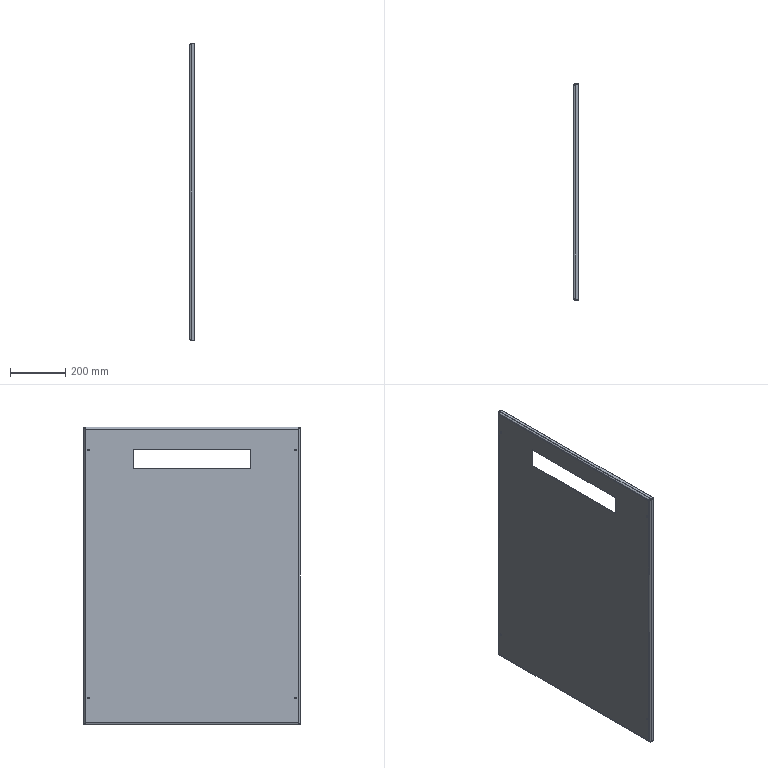Component | SolidWorks | RearLowerDoorPanel(No.28)-1 | 1 solid | 50 faces | volume 1733113 mm3 | plane 26 | cylinder 16 | spline 8 | commonest cylinder face diameters 6.5 x8 14 x4 10 x4 | material Plain Carbon Steel